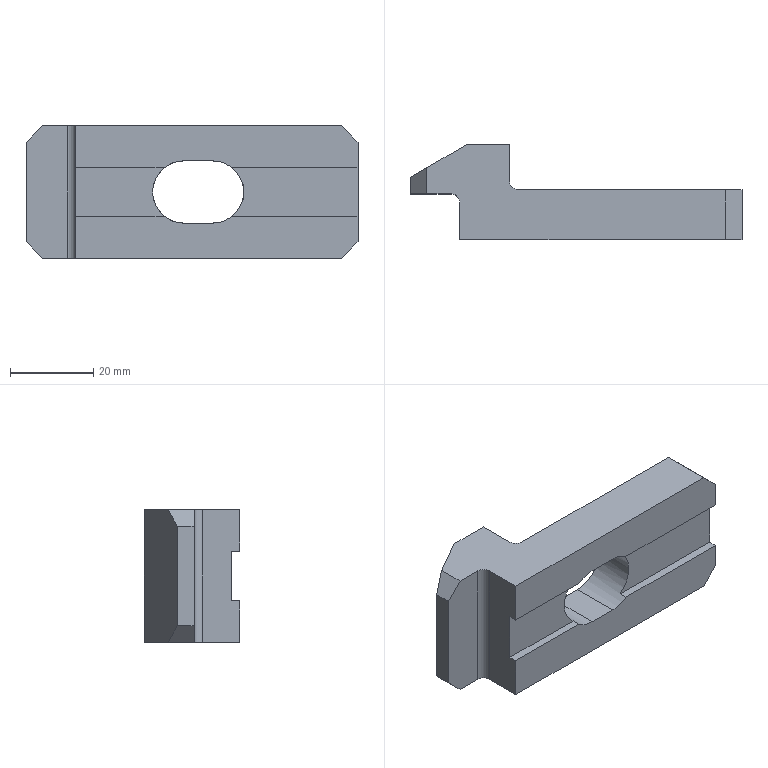Component | SolidWorks | JB_T8010.10-1999ElbowClampPlateTypeA12-1 | 1 solid | 28 faces | box 80 x 23 x 32 mm | volume 28429 mm3 | plane 24 | cylinder 4 | commonest cylinder face diameters 15 x2 4 x2 | material Nickel
STEP:
#1=COLOUR_RGB('',0.7922,0.8196,0.9333);
#2=FILL_AREA_STYLE_COLOUR('',#1);
#3=FILL_AREA_STYLE('',(#2));
#4=SURFACE_STYLE_FILL_AREA(#3);
#5=SURFACE_SIDE_STYLE('',(#4));
#6=SURFACE_STYLE_USAGE(.BOTH.,#5);
#7=PRESENTATION_STYLE_ASSIGNMENT((#6));
#8=CARTESIAN_POINT('',(2.48,8.528,-0.2362));
#9=VERTEX_POINT('',#8);
#10=CARTESIAN_POINT('',(3.327,8.528,-0.2362));
#11=VERTEX_POINT('',#10);
#12=CARTESIAN_POINT('',(2.008,8.528,-0.2362));
#13=DIRECTION('',(1.,0.,0.));
#14=VECTOR('',#13,39.37);
#15=LINE('',#12,#14);
#16=EDGE_CURVE('',#9,#11,#15,.T.);
#17=ORIENTED_EDGE('',*,*,#16,.F.);
#18=CARTESIAN_POINT('',(2.48,8.528,-0.6299));
#19=VERTEX_POINT('',#18);
#20=CARTESIAN_POINT('',(2.48,8.528,0.6299));
#21=DIRECTION('',(-0.,0.,-1.));
#22=VECTOR('',#21,39.37);
#23=LINE('',#20,#22);
#24=EDGE_CURVE('',#9,#19,#23,.T.);
#25=ORIENTED_EDGE('',*,*,#24,.T.);
#26=CARTESIAN_POINT('',(5.,8.528,-0.6299));
#27=VERTEX_POINT('',#26);
#28=CARTESIAN_POINT('',(2.48,8.528,-0.6299));
#29=DIRECTION('',(1.,0.,0.));
#30=VECTOR('',#29,39.37);
#31=LINE('',#28,#30);
#32=EDGE_CURVE('',#19,#27,#31,.T.);
#33=ORIENTED_EDGE('',*,*,#32,.T.);
#34=CARTESIAN_POINT('',(5.157,8.528,-0.4724));
#35=VERTEX_POINT('',#34);
#36=CARTESIAN_POINT('',(3.819,8.528,-1.811));
#37=DIRECTION('',(0.7071,0.,0.7071));
#38=VECTOR('',#37,39.37);
#39=LINE('',#36,#38);
#40=EDGE_CURVE('',#27,#35,#39,.T.);
#41=ORIENTED_EDGE('',*,*,#40,.T.);
#42=CARTESIAN_POINT('',(5.157,8.528,-0.2362));
#43=VERTEX_POINT('',#42);
#44=CARTESIAN_POINT('',(5.157,8.528,-0.6299));
#45=DIRECTION('',(0.,0.,1.));
#46=VECTOR('',#45,39.37);
#47=LINE('',#44,#46);
#48=EDGE_CURVE('',#35,#43,#47,.T.);
#49=ORIENTED_EDGE('',*,*,#48,.T.);
#50=CARTESIAN_POINT('',(3.957,8.528,-0.2362));
#51=VERTEX_POINT('',#50);
#52=CARTESIAN_POINT('',(2.008,8.528,-0.2362));
#53=DIRECTION('',(1.,0.,0.));
#54=VECTOR('',#53,39.37);
#55=LINE('',#52,#54);
#56=EDGE_CURVE('',#51,#43,#55,.T.);
#57=ORIENTED_EDGE('',*,*,#56,.F.);
#58=CARTESIAN_POINT('',(3.78,8.528,-0.2953));
#59=VERTEX_POINT('',#58);
#60=CARTESIAN_POINT('',(3.78,8.528,0.));
#61=DIRECTION('',(0.,-1.,0.));
#62=DIRECTION('',(0.,0.,-1.));
#63=AXIS2_PLACEMENT_3D('',#60,#61,#62);
#64=CIRCLE('',#63,0.2953);
#65=EDGE_CURVE('',#59,#51,#64,.T.);
#66=ORIENTED_EDGE('',*,*,#65,.F.);
#67=CARTESIAN_POINT('',(3.504,8.528,-0.2953));
#68=VERTEX_POINT('',#67);
#69=CARTESIAN_POINT('',(3.504,8.528,-0.2953));
#70=DIRECTION('',(1.,0.,0.));
#71=VECTOR('',#70,39.37);
#72=LINE('',#69,#71);
#73=EDGE_CURVE('',#68,#59,#72,.T.);
#74=ORIENTED_EDGE('',*,*,#73,.F.);
#75=CARTESIAN_POINT('',(3.504,8.528,0.));
#76=DIRECTION('',(0.,-1.,0.));
#77=DIRECTION('',(0.,0.,-1.));
#78=AXIS2_PLACEMENT_3D('',#75,#76,#77);
#79=CIRCLE('',#78,0.2953);
#80=EDGE_CURVE('',#11,#68,#79,.T.);
#81=ORIENTED_EDGE('',*,*,#80,.F.);
#82=EDGE_LOOP('',(#17,#25,#33,#41,#49,#57,#66,#74,#81));
#83=FACE_OUTER_BOUND('',#82,.T.);
#84=CARTESIAN_POINT('',(2.008,8.528,0.));
#85=DIRECTION('',(0.,-1.,0.));
#86=DIRECTION('',(0.,0.,-1.));
#87=AXIS2_PLACEMENT_3D('',#84,#85,#86);
#88=PLANE('',#87);
#89=ADVANCED_FACE('',(#83),#88,.T.);
#90=CARTESIAN_POINT('',(5.,9.,-0.6299));
#91=VERTEX_POINT('',#90);
#92=CARTESIAN_POINT('',(3.031,9.,-0.6299));
#93=VERTEX_POINT('',#92);
#94=CARTESIAN_POINT('',(5.157,9.,-0.6299));
#95=DIRECTION('',(-1.,0.,0.));
#96=VECTOR('',#95,39.37);
#97=LINE('',#94,#96);
#98=EDGE_CURVE('',#91,#93,#97,.T.);
#99=ORIENTED_EDGE('',*,*,#98,.F.);
#100=CARTESIAN_POINT('',(5.,8.803,-0.6299));
#101=DIRECTION('',(0.,-1.,0.));
#102=VECTOR('',#101,39.37);
#103=LINE('',#100,#102);
#104=EDGE_CURVE('',#91,#27,#103,.T.);
#105=ORIENTED_EDGE('',*,*,#104,.T.);
#106=ORIENTED_EDGE('',*,*,#32,.F.);
#107=CARTESIAN_POINT('',(2.48,8.882,-0.6299));
#108=VERTEX_POINT('',#107);
#109=CARTESIAN_POINT('',(2.48,8.961,-0.6299));
#110=DIRECTION('',(0.,-1.,0.));
#111=VECTOR('',#110,39.37);
#112=LINE('',#109,#111);
#113=EDGE_CURVE('',#108,#19,#112,.T.);
#114=ORIENTED_EDGE('',*,*,#113,.F.);
#115=CARTESIAN_POINT('',(2.402,8.961,-0.6299));
#116=VERTEX_POINT('',#115);
#117=CARTESIAN_POINT('',(2.402,8.882,-0.6299));
#118=DIRECTION('',(0.,0.,1.));
#119=DIRECTION('',(1.,0.,0.));
#120=AXIS2_PLACEMENT_3D('',#117,#118,#119);
#121=CIRCLE('',#120,0.07874);
#122=EDGE_CURVE('',#108,#116,#121,.T.);
#123=ORIENTED_EDGE('',*,*,#122,.T.);
#124=CARTESIAN_POINT('',(2.165,8.961,-0.6299));
#125=VERTEX_POINT('',#124);
#126=CARTESIAN_POINT('',(2.008,8.961,-0.6299));
#127=DIRECTION('',(1.,0.,0.));
#128=VECTOR('',#127,39.37);
#129=LINE('',#126,#128);
#130=EDGE_CURVE('',#125,#116,#129,.T.);
#131=ORIENTED_EDGE('',*,*,#130,.F.);
#132=CARTESIAN_POINT('',(2.165,9.209,-0.6299));
#133=VERTEX_POINT('',#132);
#134=CARTESIAN_POINT('',(2.165,8.803,-0.6299));
#135=DIRECTION('',(0.,1.,0.));
#136=VECTOR('',#135,39.37);
#137=LINE('',#134,#136);
#138=EDGE_CURVE('',#125,#133,#137,.T.);
#139=ORIENTED_EDGE('',*,*,#138,.T.);
#140=CARTESIAN_POINT('',(2.553,9.433,-0.6299));
#141=VERTEX_POINT('',#140);
#142=CARTESIAN_POINT('',(1.871,9.04,-0.6299));
#143=DIRECTION('',(0.866,0.5,0.));
#144=VECTOR('',#143,39.37);
#145=LINE('',#142,#144);
#146=EDGE_CURVE('',#133,#141,#145,.T.);
#147=ORIENTED_EDGE('',*,*,#146,.T.);
#148=CARTESIAN_POINT('',(2.953,9.433,-0.6299));
#149=VERTEX_POINT('',#148);
#150=CARTESIAN_POINT('',(2.953,9.433,-0.6299));
#151=DIRECTION('',(-1.,0.,0.));
#152=VECTOR('',#151,39.37);
#153=LINE('',#150,#152);
#154=EDGE_CURVE('',#149,#141,#153,.T.);
#155=ORIENTED_EDGE('',*,*,#154,.F.);
#156=CARTESIAN_POINT('',(2.953,9.079,-0.6299));
#157=VERTEX_POINT('',#156);
#158=CARTESIAN_POINT('',(2.953,9.433,-0.6299));
#159=DIRECTION('',(0.,-1.,0.));
#160=VECTOR('',#159,39.37);
#161=LINE('',#158,#160);
#162=EDGE_CURVE('',#149,#157,#161,.T.);
#163=ORIENTED_EDGE('',*,*,#162,.T.);
#164=CARTESIAN_POINT('',(3.031,9.079,-0.6299));
#165=DIRECTION('',(0.,0.,1.));
#166=DIRECTION('',(1.,0.,0.));
#167=AXIS2_PLACEMENT_3D('',#164,#165,#166);
#168=CIRCLE('',#167,0.07874);
#169=EDGE_CURVE('',#157,#93,#168,.T.);
#170=ORIENTED_EDGE('',*,*,#169,.T.);
#171=EDGE_LOOP('',(#99,#105,#106,#114,#123,#131,#139,#147,#155,#163,#170));
#172=FACE_OUTER_BOUND('',#171,.T.);
#173=CARTESIAN_POINT('',(2.008,8.803,-0.6299));
#174=DIRECTION('',(0.,0.,1.));
#175=DIRECTION('',(1.,0.,0.));
#176=AXIS2_PLACEMENT_3D('',#173,#174,#175);
#177=PLANE('',#176);
#178=ADVANCED_FACE('',(#172),#177,.F.);
#179=CARTESIAN_POINT('',(2.553,9.433,0.6299));
#180=VERTEX_POINT('',#179);
#181=CARTESIAN_POINT('',(2.165,9.209,0.6299));
#182=VERTEX_POINT('',#181);
#183=CARTESIAN_POINT('',(1.871,9.04,0.6299));
#184=DIRECTION('',(-0.866,-0.5,0.));
#185=VECTOR('',#184,39.37);
#186=LINE('',#183,#185);
#187=EDGE_CURVE('',#180,#182,#186,.T.);
#188=ORIENTED_EDGE('',*,*,#187,.T.);
#189=CARTESIAN_POINT('',(2.165,8.961,0.6299));
#190=VERTEX_POINT('',#189);
#191=CARTESIAN_POINT('',(2.165,8.803,0.6299));
#192=DIRECTION('',(0.,-1.,0.));
#193=VECTOR('',#192,39.37);
#194=LINE('',#191,#193);
#195=EDGE_CURVE('',#182,#190,#194,.T.);
#196=ORIENTED_EDGE('',*,*,#195,.T.);
#197=CARTESIAN_POINT('',(2.402,8.961,0.6299));
#198=VERTEX_POINT('',#197);
#199=CARTESIAN_POINT('',(2.48,8.961,0.6299));
#200=DIRECTION('',(-1.,0.,0.));
#201=VECTOR('',#200,39.37);
#202=LINE('',#199,#201);
#203=EDGE_CURVE('',#198,#190,#202,.T.);
#204=ORIENTED_EDGE('',*,*,#203,.F.);
#205=CARTESIAN_POINT('',(2.48,8.882,0.6299));
#206=VERTEX_POINT('',#205);
#207=CARTESIAN_POINT('',(2.402,8.882,0.6299));
#208=DIRECTION('',(0.,0.,-1.));
#209=DIRECTION('',(-1.,0.,0.));
#210=AXIS2_PLACEMENT_3D('',#207,#208,#209);
#211=CIRCLE('',#210,0.07874);
#212=EDGE_CURVE('',#198,#206,#211,.T.);
#213=ORIENTED_EDGE('',*,*,#212,.T.);
#214=CARTESIAN_POINT('',(2.48,8.528,0.6299));
#215=VERTEX_POINT('',#214);
#216=CARTESIAN_POINT('',(2.48,8.961,0.6299));
#217=DIRECTION('',(0.,-1.,0.));
#218=VECTOR('',#217,39.37);
#219=LINE('',#216,#218);
#220=EDGE_CURVE('',#206,#215,#219,.T.);
#221=ORIENTED_EDGE('',*,*,#220,.T.);
#222=CARTESIAN_POINT('',(5.,8.528,0.6299));
#223=VERTEX_POINT('',#222);
#224=CARTESIAN_POINT('',(5.157,8.528,0.6299));
#225=DIRECTION('',(-1.,0.,0.));
#226=VECTOR('',#225,39.37);
#227=LINE('',#224,#226);
#228=EDGE_CURVE('',#223,#215,#227,.T.);
#229=ORIENTED_EDGE('',*,*,#228,.F.);
#230=CARTESIAN_POINT('',(5.,9.,0.6299));
#231=VERTEX_POINT('',#230);
#232=CARTESIAN_POINT('',(5.,8.803,0.6299));
#233=DIRECTION('',(0.,1.,0.));
#234=VECTOR('',#233,39.37);
#235=LINE('',#232,#234);
#236=EDGE_CURVE('',#223,#231,#235,.T.);
#237=ORIENTED_EDGE('',*,*,#236,.T.);
#238=CARTESIAN_POINT('',(3.031,9.,0.6299));
#239=VERTEX_POINT('',#238);
#240=CARTESIAN_POINT('',(5.157,9.,0.6299));
#241=DIRECTION('',(1.,0.,0.));
#242=VECTOR('',#241,39.37);
#243=LINE('',#240,#242);
#244=EDGE_CURVE('',#239,#231,#243,.T.);
#245=ORIENTED_EDGE('',*,*,#244,.F.);
#246=CARTESIAN_POINT('',(2.953,9.079,0.6299));
#247=VERTEX_POINT('',#246);
#248=CARTESIAN_POINT('',(3.031,9.079,0.6299));
#249=DIRECTION('',(0.,0.,-1.));
#250=DIRECTION('',(-1.,0.,0.));
#251=AXIS2_PLACEMENT_3D('',#248,#249,#250);
#252=CIRCLE('',#251,0.07874);
#253=EDGE_CURVE('',#239,#247,#252,.T.);
#254=ORIENTED_EDGE('',*,*,#253,.T.);
#255=CARTESIAN_POINT('',(2.953,9.433,0.6299));
#256=VERTEX_POINT('',#255);
#257=CARTESIAN_POINT('',(2.953,9.433,0.6299));
#258=DIRECTION('',(0.,-1.,0.));
#259=VECTOR('',#258,39.37);
#260=LINE('',#257,#259);
#261=EDGE_CURVE('',#256,#247,#260,.T.);
#262=ORIENTED_EDGE('',*,*,#261,.F.);
#263=CARTESIAN_POINT('',(2.008,9.433,0.6299));
#264=DIRECTION('',(1.,0.,0.));
#265=VECTOR('',#264,39.37);
#266=LINE('',#263,#265);
#267=EDGE_CURVE('',#180,#256,#266,.T.);
#268=ORIENTED_EDGE('',*,*,#267,.F.);
#269=EDGE_LOOP('',(#188,#196,#204,#213,#221,#229,#237,#245,#254,#262,#268));
#270=FACE_OUTER_BOUND('',#269,.T.);
#271=CARTESIAN_POINT('',(2.008,8.803,0.6299));
#272=DIRECTION('',(0.,0.,-1.));
#273=DIRECTION('',(-1.,0.,0.));
#274=AXIS2_PLACEMENT_3D('',#271,#272,#273);
#275=PLANE('',#274);
#276=ADVANCED_FACE('',(#270),#275,.F.);
#277=CARTESIAN_POINT('',(5.157,8.607,-0.2362));
#278=VERTEX_POINT('',#277);
#279=CARTESIAN_POINT('',(5.157,8.607,0.2362));
#280=VERTEX_POINT('',#279);
#281=CARTESIAN_POINT('',(5.157,8.607,-0.6299));
#282=DIRECTION('',(0.,0.,1.));
#283=VECTOR('',#282,39.37);
#284=LINE('',#281,#283);
#285=EDGE_CURVE('',#278,#280,#284,.T.);
#286=ORIENTED_EDGE('',*,*,#285,.F.);
#287=CARTESIAN_POINT('',(5.157,8.803,-0.2362));
#288=DIRECTION('',(0.,-1.,0.));
#289=VECTOR('',#288,39.37);
#290=LINE('',#287,#289);
#291=EDGE_CURVE('',#278,#43,#290,.T.);
#292=ORIENTED_EDGE('',*,*,#291,.T.);
#293=ORIENTED_EDGE('',*,*,#48,.F.);
#294=CARTESIAN_POINT('',(5.157,9.,-0.4724));
#295=VERTEX_POINT('',#294);
#296=CARTESIAN_POINT('',(5.157,8.803,-0.4724));
#297=DIRECTION('',(0.,1.,0.));
#298=VECTOR('',#297,39.37);
#299=LINE('',#296,#298);
#300=EDGE_CURVE('',#35,#295,#299,.T.);
#301=ORIENTED_EDGE('',*,*,#300,.T.);
#302=CARTESIAN_POINT('',(5.157,9.,0.4724));
#303=VERTEX_POINT('',#302);
#304=CARTESIAN_POINT('',(5.157,9.,-0.6299));
#305=DIRECTION('',(0.,0.,-1.));
#306=VECTOR('',#305,39.37);
#307=LINE('',#304,#306);
#308=EDGE_CURVE('',#303,#295,#307,.T.);
#309=ORIENTED_EDGE('',*,*,#308,.F.);
#310=CARTESIAN_POINT('',(5.157,8.528,0.4724));
#311=VERTEX_POINT('',#310);
#312=CARTESIAN_POINT('',(5.157,8.803,0.4724));
#313=DIRECTION('',(0.,-1.,0.));
#314=VECTOR('',#313,39.37);
#315=LINE('',#312,#314);
#316=EDGE_CURVE('',#303,#311,#315,.T.);
#317=ORIENTED_EDGE('',*,*,#316,.T.);
#318=CARTESIAN_POINT('',(5.157,8.528,0.2362));
#319=VERTEX_POINT('',#318);
#320=CARTESIAN_POINT('',(5.157,8.528,-0.6299));
#321=DIRECTION('',(0.,0.,1.));
#322=VECTOR('',#321,39.37);
#323=LINE('',#320,#322);
#324=EDGE_CURVE('',#319,#311,#323,.T.);
#325=ORIENTED_EDGE('',*,*,#324,.F.);
#326=CARTESIAN_POINT('',(5.157,8.803,0.2362));
#327=DIRECTION('',(0.,1.,0.));
#328=VECTOR('',#327,39.37);
#329=LINE('',#326,#328);
#330=EDGE_CURVE('',#319,#280,#329,.T.);
#331=ORIENTED_EDGE('',*,*,#330,.T.);
#332=EDGE_LOOP('',(#286,#292,#293,#301,#309,#317,#325,#331));
#333=FACE_OUTER_BOUND('',#332,.T.);
#334=CARTESIAN_POINT('',(5.157,8.803,-0.6299));
#335=DIRECTION('',(-1.,0.,0.));
#336=DIRECTION('',(0.,0.,1.));
#337=AXIS2_PLACEMENT_3D('',#334,#335,#336);
#338=PLANE('',#337);
#339=ADVANCED_FACE('',(#333),#338,.F.);
#340=CARTESIAN_POINT('',(3.327,8.607,-0.2362));
#341=VERTEX_POINT('',#340);
#342=CARTESIAN_POINT('',(3.327,8.803,-0.2362));
#343=DIRECTION('',(0.,1.,0.));
#344=VECTOR('',#343,39.37);
#345=LINE('',#342,#344);
#346=EDGE_CURVE('',#11,#341,#345,.T.);
#347=ORIENTED_EDGE('',*,*,#346,.F.);
#348=ORIENTED_EDGE('',*,*,#80,.T.);
#349=CARTESIAN_POINT('',(3.504,9.,-0.2953));
#350=VERTEX_POINT('',#349);
#351=CARTESIAN_POINT('',(3.504,8.803,-0.2953));
#352=DIRECTION('',(0.,-1.,0.));
#353=VECTOR('',#352,39.37);
#354=LINE('',#351,#353);
#355=EDGE_CURVE('',#350,#68,#354,.T.);
#356=ORIENTED_EDGE('',*,*,#355,.F.);
#357=CARTESIAN_POINT('',(3.504,9.,0.2953));
#358=VERTEX_POINT('',#357);
#359=CARTESIAN_POINT('',(3.504,9.,0.));
#360=DIRECTION('',(0.,1.,0.));
#361=DIRECTION('',(0.,0.,-1.));
#362=AXIS2_PLACEMENT_3D('',#359,#360,#361);
#363=CIRCLE('',#362,0.2953);
#364=EDGE_CURVE('',#350,#358,#363,.T.);
#365=ORIENTED_EDGE('',*,*,#364,.T.);
#366=CARTESIAN_POINT('',(3.504,8.528,0.2953));
#367=VERTEX_POINT('',#366);
#368=CARTESIAN_POINT('',(3.504,8.803,0.2953));
#369=DIRECTION('',(0.,-1.,0.));
#370=VECTOR('',#369,39.37);
#371=LINE('',#368,#370);
#372=EDGE_CURVE('',#358,#367,#371,.T.);
#373=ORIENTED_EDGE('',*,*,#372,.T.);
#374=CARTESIAN_POINT('',(3.327,8.528,0.2362));
#375=VERTEX_POINT('',#374);
#376=CARTESIAN_POINT('',(3.504,8.528,0.));
#377=DIRECTION('',(0.,-1.,0.));
#378=DIRECTION('',(0.,0.,-1.));
#379=AXIS2_PLACEMENT_3D('',#376,#377,#378);
#380=CIRCLE('',#379,0.2953);
#381=EDGE_CURVE('',#367,#375,#380,.T.);
#382=ORIENTED_EDGE('',*,*,#381,.T.);
#383=CARTESIAN_POINT('',(3.327,8.607,0.2362));
#384=VERTEX_POINT('',#383);
#385=CARTESIAN_POINT('',(3.327,8.803,0.2362));
#386=DIRECTION('',(0.,-1.,0.));
#387=VECTOR('',#386,39.37);
#388=LINE('',#385,#387);
#389=EDGE_CURVE('',#384,#375,#388,.T.);
#390=ORIENTED_EDGE('',*,*,#389,.F.);
#391=CARTESIAN_POINT('',(3.504,8.607,0.));
#392=DIRECTION('',(0.,-1.,0.));
#393=DIRECTION('',(0.,0.,-1.));
#394=AXIS2_PLACEMENT_3D('',#391,#392,#393);
#395=CIRCLE('',#394,0.2953);
#396=EDGE_CURVE('',#384,#341,#395,.T.);
#397=ORIENTED_EDGE('',*,*,#396,.T.);
#398=EDGE_LOOP('',(#347,#348,#356,#365,#373,#382,#390,#397));
#399=FACE_OUTER_BOUND('',#398,.T.);
#400=CARTESIAN_POINT('',(3.504,8.803,0.));
#401=DIRECTION('',(0.,-1.,0.));
#402=DIRECTION('',(0.,0.,-1.));
#403=AXIS2_PLACEMENT_3D('',#400,#401,#402);
#404=CYLINDRICAL_SURFACE('',#403,0.2953);
#405=ADVANCED_FACE('',(#399),#404,.F.);
#406=CARTESIAN_POINT('',(3.78,9.,0.2953));
#407=VERTEX_POINT('',#406);
#408=CARTESIAN_POINT('',(3.78,8.528,0.2953));
#409=VERTEX_POINT('',#408);
#410=CARTESIAN_POINT('',(3.78,8.803,0.2953));
#411=DIRECTION('',(0.,-1.,0.));
#412=VECTOR('',#411,39.37);
#413=LINE('',#410,#412);
#414=EDGE_CURVE('',#407,#409,#413,.T.);
#415=ORIENTED_EDGE('',*,*,#414,.T.);
#416=CARTESIAN_POINT('',(3.504,8.528,0.2953));
#417=DIRECTION('',(-1.,0.,0.));
#418=VECTOR('',#417,39.37);
#419=LINE('',#416,#418);
#420=EDGE_CURVE('',#409,#367,#419,.T.);
#421=ORIENTED_EDGE('',*,*,#420,.T.);
#422=ORIENTED_EDGE('',*,*,#372,.F.);
#423=CARTESIAN_POINT('',(5.157,9.,0.2953));
#424=DIRECTION('',(1.,0.,0.));
#425=VECTOR('',#424,39.37);
#426=LINE('',#423,#425);
#427=EDGE_CURVE('',#358,#407,#426,.T.);
#428=ORIENTED_EDGE('',*,*,#427,.T.);
#429=EDGE_LOOP('',(#415,#421,#422,#428));
#430=FACE_OUTER_BOUND('',#429,.T.);
#431=CARTESIAN_POINT('',(3.504,8.803,0.2953));
#432=DIRECTION('',(0.,0.,-1.));
#433=DIRECTION('',(-1.,0.,0.));
#434=AXIS2_PLACEMENT_3D('',#431,#432,#433);
#435=PLANE('',#434);
#436=ADVANCED_FACE('',(#430),#435,.T.);
#437=CARTESIAN_POINT('',(3.957,8.607,-0.2362));
#438=VERTEX_POINT('',#437);
#439=CARTESIAN_POINT('',(3.957,8.803,-0.2362));
#440=DIRECTION('',(0.,-1.,0.));
#441=VECTOR('',#440,39.37);
#442=LINE('',#439,#441);
#443=EDGE_CURVE('',#438,#51,#442,.T.);
#444=ORIENTED_EDGE('',*,*,#443,.F.);
#445=CARTESIAN_POINT('',(3.957,8.607,0.2362));
#446=VERTEX_POINT('',#445);
#447=CARTESIAN_POINT('',(3.78,8.607,0.));
#448=DIRECTION('',(0.,-1.,0.));
#449=DIRECTION('',(0.,0.,-1.));
#450=AXIS2_PLACEMENT_3D('',#447,#448,#449);
#451=CIRCLE('',#450,0.2953);
#452=EDGE_CURVE('',#438,#446,#451,.T.);
#453=ORIENTED_EDGE('',*,*,#452,.T.);
#454=CARTESIAN_POINT('',(3.957,8.528,0.2362));
#455=VERTEX_POINT('',#454);
#456=CARTESIAN_POINT('',(3.957,8.803,0.2362));
#457=DIRECTION('',(0.,1.,0.));
#458=VECTOR('',#457,39.37);
#459=LINE('',#456,#458);
#460=EDGE_CURVE('',#455,#446,#459,.T.);
#461=ORIENTED_EDGE('',*,*,#460,.F.);
#462=CARTESIAN_POINT('',(3.78,8.528,0.));
#463=DIRECTION('',(0.,-1.,0.));
#464=DIRECTION('',(0.,0.,-1.));
#465=AXIS2_PLACEMENT_3D('',#462,#463,#464);
#466=CIRCLE('',#465,0.2953);
#467=EDGE_CURVE('',#455,#409,#466,.T.);
#468=ORIENTED_EDGE('',*,*,#467,.T.);
#469=ORIENTED_EDGE('',*,*,#414,.F.);
#470=CARTESIAN_POINT('',(3.78,9.,-0.2953));
#471=VERTEX_POINT('',#470);
#472=CARTESIAN_POINT('',(3.78,9.,0.));
#473=DIRECTION('',(0.,1.,0.));
#474=DIRECTION('',(0.,0.,-1.));
#475=AXIS2_PLACEMENT_3D('',#472,#473,#474);
#476=CIRCLE('',#475,0.2953);
#477=EDGE_CURVE('',#407,#471,#476,.T.);
#478=ORIENTED_EDGE('',*,*,#477,.T.);
#479=CARTESIAN_POINT('',(3.78,8.803,-0.2953));
#480=DIRECTION('',(0.,-1.,0.));
#481=VECTOR('',#480,39.37);
#482=LINE('',#479,#481);
#483=EDGE_CURVE('',#471,#59,#482,.T.);
#484=ORIENTED_EDGE('',*,*,#483,.T.);
#485=ORIENTED_EDGE('',*,*,#65,.T.);
#486=EDGE_LOOP('',(#444,#453,#461,#468,#469,#478,#484,#485));
#487=FACE_OUTER_BOUND('',#486,.T.);
#488=CARTESIAN_POINT('',(3.78,8.803,0.));
#489=DIRECTION('',(0.,-1.,0.));
#490=DIRECTION('',(0.,0.,-1.));
#491=AXIS2_PLACEMENT_3D('',#488,#489,#490);
#492=CYLINDRICAL_SURFACE('',#491,0.2953);
#493=ADVANCED_FACE('',(#487),#492,.F.);
#494=ORIENTED_EDGE('',*,*,#355,.T.);
#495=ORIENTED_EDGE('',*,*,#73,.T.);
#496=ORIENTED_EDGE('',*,*,#483,.F.);
#497=CARTESIAN_POINT('',(5.157,9.,-0.2953));
#498=DIRECTION('',(-1.,0.,0.));
#499=VECTOR('',#498,39.37);
#500=LINE('',#497,#499);
#501=EDGE_CURVE('',#471,#350,#500,.T.);
#502=ORIENTED_EDGE('',*,*,#501,.T.);
#503=EDGE_LOOP('',(#494,#495,#496,#502));
#504=FACE_OUTER_BOUND('',#503,.T.);
#505=CARTESIAN_POINT('',(3.504,8.803,-0.2953));
#506=DIRECTION('',(0.,0.,1.));
#507=DIRECTION('',(1.,0.,0.));
#508=AXIS2_PLACEMENT_3D('',#505,#506,#507);
#509=PLANE('',#508);
#510=ADVANCED_FACE('',(#504),#509,.T.);
#511=ORIENTED_EDGE('',*,*,#24,.F.);
#512=CARTESIAN_POINT('',(2.48,8.607,-0.2362));
#513=VERTEX_POINT('',#512);
#514=CARTESIAN_POINT('',(2.48,8.961,-0.2362));
#515=DIRECTION('',(0.,1.,0.));
#516=VECTOR('',#515,39.37);
#517=LINE('',#514,#516);
#518=EDGE_CURVE('',#9,#513,#517,.T.);
#519=ORIENTED_EDGE('',*,*,#518,.T.);
#520=CARTESIAN_POINT('',(2.48,8.607,0.2362));
#521=VERTEX_POINT('',#520);
#522=CARTESIAN_POINT('',(2.48,8.607,-0.6299));
#523=DIRECTION('',(-0.,0.,-1.));
#524=VECTOR('',#523,39.37);
#525=LINE('',#522,#524);
#526=EDGE_CURVE('',#521,#513,#525,.T.);
#527=ORIENTED_EDGE('',*,*,#526,.F.);
#528=CARTESIAN_POINT('',(2.48,8.528,0.2362));
#529=VERTEX_POINT('',#528);
#530=CARTESIAN_POINT('',(2.48,8.961,0.2362));
#531=DIRECTION('',(0.,-1.,0.));
#532=VECTOR('',#531,39.37);
#533=LINE('',#530,#532);
#534=EDGE_CURVE('',#521,#529,#533,.T.);
#535=ORIENTED_EDGE('',*,*,#534,.T.);
#536=CARTESIAN_POINT('',(2.48,8.528,0.6299));
#537=DIRECTION('',(-0.,0.,-1.));
#538=VECTOR('',#537,39.37);
#539=LINE('',#536,#538);
#540=EDGE_CURVE('',#215,#529,#539,.T.);
#541=ORIENTED_EDGE('',*,*,#540,.F.);
#542=ORIENTED_EDGE('',*,*,#220,.F.);
#543=CARTESIAN_POINT('',(2.48,8.882,-0.6299));
#544=DIRECTION('',(-0.,0.,-1.));
#545=VECTOR('',#544,39.37);
#546=LINE('',#543,#545);
#547=EDGE_CURVE('',#206,#108,#546,.T.);
#548=ORIENTED_EDGE('',*,*,#547,.T.);
#549=ORIENTED_EDGE('',*,*,#113,.T.);
#550=EDGE_LOOP('',(#511,#519,#527,#535,#541,#542,#548,#549));
#551=FACE_OUTER_BOUND('',#550,.T.);
#552=CARTESIAN_POINT('',(2.48,8.961,-0.6299));
#553=DIRECTION('',(1.,0.,-0.));
#554=DIRECTION('',(-0.,0.,-1.));
#555=AXIS2_PLACEMENT_3D('',#552,#553,#554);
#556=PLANE('',#555);
#557=ADVANCED_FACE('',(#551),#556,.F.);
#558=CARTESIAN_POINT('',(2.008,8.961,0.4724));
#559=VERTEX_POINT('',#558);
#560=CARTESIAN_POINT('',(2.008,8.961,-0.4724));
#561=VERTEX_POINT('',#560);
#562=CARTESIAN_POINT('',(2.008,8.961,0.6299));
#563=DIRECTION('',(0.,0.,-1.));
#564=VECTOR('',#563,39.37);
#565=LINE('',#562,#564);
#566=EDGE_CURVE('',#559,#561,#565,.T.);
#567=ORIENTED_EDGE('',*,*,#566,.F.);
#568=CARTESIAN_POINT('',(2.008,9.118,0.4724));
#569=VERTEX_POINT('',#568);
#570=CARTESIAN_POINT('',(2.008,8.803,0.4724));
#571=DIRECTION('',(0.,1.,0.));
#572=VECTOR('',#571,39.37);
#573=LINE('',#570,#572);
#574=EDGE_CURVE('',#559,#569,#573,.T.);
#575=ORIENTED_EDGE('',*,*,#574,.T.);
#576=CARTESIAN_POINT('',(2.008,9.118,-0.4724));
#577=VERTEX_POINT('',#576);
#578=CARTESIAN_POINT('',(2.008,9.118,-0.6299));
#579=DIRECTION('',(0.,0.,1.));
#580=VECTOR('',#579,39.37);
#581=LINE('',#578,#580);
#582=EDGE_CURVE('',#577,#569,#581,.T.);
#583=ORIENTED_EDGE('',*,*,#582,.F.);
#584=CARTESIAN_POINT('',(2.008,8.803,-0.4724));
#585=DIRECTION('',(0.,-1.,0.));
#586=VECTOR('',#585,39.37);
#587=LINE('',#584,#586);
#588=EDGE_CURVE('',#577,#561,#587,.T.);
#589=ORIENTED_EDGE('',*,*,#588,.T.);
#590=EDGE_LOOP('',(#567,#575,#583,#589));
#591=FACE_OUTER_BOUND('',#590,.T.);
#592=CARTESIAN_POINT('',(2.008,8.803,0.6299));
#593=DIRECTION('',(1.,0.,0.));
#594=DIRECTION('',(0.,0.,-1.));
#595=AXIS2_PLACEMENT_3D('',#592,#593,#594);
#596=PLANE('',#595);
#597=ADVANCED_FACE('',(#591),#596,.F.);
#598=ORIENTED_EDGE('',*,*,#364,.F.);
#599=ORIENTED_EDGE('',*,*,#501,.F.);
#600=ORIENTED_EDGE('',*,*,#477,.F.);
#601=ORIENTED_EDGE('',*,*,#427,.F.);
#602=EDGE_LOOP('',(#598,#599,#600,#601));
#603=FACE_BOUND('',#602,.T.);
#604=ORIENTED_EDGE('',*,*,#244,.T.);
#605=CARTESIAN_POINT('',(5.157,9.,0.4724));
#606=DIRECTION('',(0.7071,0.,-0.7071));
#607=VECTOR('',#606,39.37);
#608=LINE('',#605,#607);
#609=EDGE_CURVE('',#231,#303,#608,.T.);
#610=ORIENTED_EDGE('',*,*,#609,.T.);
#611=ORIENTED_EDGE('',*,*,#308,.T.);
#612=CARTESIAN_POINT('',(5.,9.,-0.6299));
#613=DIRECTION('',(-0.7071,0.,-0.7071));
#614=VECTOR('',#613,39.37);
#615=LINE('',#612,#614);
#616=EDGE_CURVE('',#295,#91,#615,.T.);
#617=ORIENTED_EDGE('',*,*,#616,.T.);
#618=ORIENTED_EDGE('',*,*,#98,.T.);
#619=CARTESIAN_POINT('',(3.031,9.,0.6299));
#620=DIRECTION('',(0.,0.,1.));
#621=VECTOR('',#620,39.37);
#622=LINE('',#619,#621);
#623=EDGE_CURVE('',#93,#239,#622,.T.);
#624=ORIENTED_EDGE('',*,*,#623,.T.);
#625=EDGE_LOOP('',(#604,#610,#611,#617,#618,#624));
#626=FACE_OUTER_BOUND('',#625,.T.);
#627=CARTESIAN_POINT('',(5.157,9.,-0.6299));
#628=DIRECTION('',(0.,-1.,0.));
#629=DIRECTION('',(0.,0.,-1.));
#630=AXIS2_PLACEMENT_3D('',#627,#628,#629);
#631=PLANE('',#630);
#632=ADVANCED_FACE('',(#603,#626),#631,.F.);
#633=ORIENTED_EDGE('',*,*,#261,.T.);
#634=CARTESIAN_POINT('',(2.953,9.079,-0.6299));
#635=DIRECTION('',(-0.,0.,-1.));
#636=VECTOR('',#635,39.37);
#637=LINE('',#634,#636);
#638=EDGE_CURVE('',#247,#157,#637,.T.);
#639=ORIENTED_EDGE('',*,*,#638,.T.);
#640=ORIENTED_EDGE('',*,*,#162,.F.);
#641=CARTESIAN_POINT('',(2.953,9.433,0.6299));
#642=DIRECTION('',(-0.,0.,-1.));
#643=VECTOR('',#642,39.37);
#644=LINE('',#641,#643);
#645=EDGE_CURVE('',#256,#149,#644,.T.);
#646=ORIENTED_EDGE('',*,*,#645,.F.);
#647=EDGE_LOOP('',(#633,#639,#640,#646));
#648=FACE_OUTER_BOUND('',#647,.T.);
#649=CARTESIAN_POINT('',(2.953,9.433,0.6299));
#650=DIRECTION('',(-1.,0.,0.));
#651=DIRECTION('',(0.,0.,1.));
#652=AXIS2_PLACEMENT_3D('',#649,#650,#651);
#653=PLANE('',#652);
#654=ADVANCED_FACE('',(#648),#653,.F.);
#655=CARTESIAN_POINT('',(2.553,9.433,-0.6299));
#656=DIRECTION('',(0.,0.,-1.));
#657=VECTOR('',#656,39.37);
#658=LINE('',#655,#657);
#659=EDGE_CURVE('',#180,#141,#658,.T.);
#660=ORIENTED_EDGE('',*,*,#659,.F.);
#661=ORIENTED_EDGE('',*,*,#267,.T.);
#662=ORIENTED_EDGE('',*,*,#645,.T.);
#663=ORIENTED_EDGE('',*,*,#154,.T.);
#664=EDGE_LOOP('',(#660,#661,#662,#663));
#665=FACE_OUTER_BOUND('',#664,.T.);
#666=CARTESIAN_POINT('',(2.008,9.433,-0.6299));
#667=DIRECTION('',(0.,1.,0.));
#668=DIRECTION('',(0.,0.,1.));
#669=AXIS2_PLACEMENT_3D('',#666,#667,#668);
#670=PLANE('',#669);
#671=ADVANCED_FACE('',(#665),#670,.T.);
#672=ORIENTED_EDGE('',*,*,#203,.T.);
#673=CARTESIAN_POINT('',(2.087,8.961,0.5512));
#674=DIRECTION('',(-0.7071,0.,-0.7071));
#675=VECTOR('',#674,39.37);
#676=LINE('',#673,#675);
#677=EDGE_CURVE('',#190,#559,#676,.T.);
#678=ORIENTED_EDGE('',*,*,#677,.T.);
#679=ORIENTED_EDGE('',*,*,#566,.T.);
#680=CARTESIAN_POINT('',(1.457,8.961,0.07874));
#681=DIRECTION('',(0.7071,0.,-0.7071));
#682=VECTOR('',#681,39.37);
#683=LINE('',#680,#682);
#684=EDGE_CURVE('',#561,#125,#683,.T.);
#685=ORIENTED_EDGE('',*,*,#684,.T.);
#686=ORIENTED_EDGE('',*,*,#130,.T.);
#687=CARTESIAN_POINT('',(2.402,8.961,0.6299));
#688=DIRECTION('',(0.,0.,1.));
#689=VECTOR('',#688,39.37);
#690=LINE('',#687,#689);
#691=EDGE_CURVE('',#116,#198,#690,.T.);
#692=ORIENTED_EDGE('',*,*,#691,.T.);
#693=EDGE_LOOP('',(#672,#678,#679,#685,#686,#692));
#694=FACE_OUTER_BOUND('',#693,.T.);
#695=CARTESIAN_POINT('',(2.008,8.961,0.6299));
#696=DIRECTION('',(0.,-1.,0.));
#697=DIRECTION('',(0.,0.,-1.));
#698=AXIS2_PLACEMENT_3D('',#695,#696,#697);
#699=PLANE('',#698);
#700=ADVANCED_FACE('',(#694),#699,.T.);
#701=ORIENTED_EDGE('',*,*,#582,.T.);
#702=CARTESIAN_POINT('',(2.065,9.151,0.5295));
#703=DIRECTION('',(0.6547,0.378,0.6547));
#704=VECTOR('',#703,39.37);
#705=LINE('',#702,#704);
#706=EDGE_CURVE('',#569,#182,#705,.T.);
#707=ORIENTED_EDGE('',*,*,#706,.T.);
#708=ORIENTED_EDGE('',*,*,#187,.F.);
#709=ORIENTED_EDGE('',*,*,#659,.T.);
#710=ORIENTED_EDGE('',*,*,#146,.F.);
#711=CARTESIAN_POINT('',(1.93,9.073,-0.3945));
#712=DIRECTION('',(-0.6547,-0.378,0.6547));
#713=VECTOR('',#712,39.37);
#714=LINE('',#711,#713);
#715=EDGE_CURVE('',#133,#577,#714,.T.);
#716=ORIENTED_EDGE('',*,*,#715,.T.);
#717=EDGE_LOOP('',(#701,#707,#708,#709,#710,#716));
#718=FACE_OUTER_BOUND('',#717,.T.);
#719=CARTESIAN_POINT('',(2.008,9.118,-0.6299));
#720=DIRECTION('',(0.5,-0.866,0.));
#721=DIRECTION('',(0.866,0.5,0.));
#722=AXIS2_PLACEMENT_3D('',#719,#720,#721);
#723=PLANE('',#722);
#724=ADVANCED_FACE('',(#718),#723,.F.);
#725=CARTESIAN_POINT('',(2.008,8.528,0.2362));
#726=DIRECTION('',(-1.,0.,-0.));
#727=VECTOR('',#726,39.37);
#728=LINE('',#725,#727);
#729=EDGE_CURVE('',#319,#455,#728,.T.);
#730=ORIENTED_EDGE('',*,*,#729,.F.);
#731=ORIENTED_EDGE('',*,*,#324,.T.);
#732=CARTESIAN_POINT('',(3.819,8.528,1.811));
#733=DIRECTION('',(-0.7071,0.,0.7071));
#734=VECTOR('',#733,39.37);
#735=LINE('',#732,#734);
#736=EDGE_CURVE('',#311,#223,#735,.T.);
#737=ORIENTED_EDGE('',*,*,#736,.T.);
#738=ORIENTED_EDGE('',*,*,#228,.T.);
#739=ORIENTED_EDGE('',*,*,#540,.T.);
#740=CARTESIAN_POINT('',(2.008,8.528,0.2362));
#741=DIRECTION('',(-1.,0.,-0.));
#742=VECTOR('',#741,39.37);
#743=LINE('',#740,#742);
#744=EDGE_CURVE('',#375,#529,#743,.T.);
#745=ORIENTED_EDGE('',*,*,#744,.F.);
#746=ORIENTED_EDGE('',*,*,#381,.F.);
#747=ORIENTED_EDGE('',*,*,#420,.F.);
#748=ORIENTED_EDGE('',*,*,#467,.F.);
#749=EDGE_LOOP('',(#730,#731,#737,#738,#739,#745,#746,#747,#748));
#750=FACE_OUTER_BOUND('',#749,.T.);
#751=CARTESIAN_POINT('',(2.008,8.528,0.));
#752=DIRECTION('',(0.,-1.,0.));
#753=DIRECTION('',(0.,0.,-1.));
#754=AXIS2_PLACEMENT_3D('',#751,#752,#753);
#755=PLANE('',#754);
#756=ADVANCED_FACE('',(#750),#755,.T.);
#757=ORIENTED_EDGE('',*,*,#253,.F.);
#758=ORIENTED_EDGE('',*,*,#623,.F.);
#759=ORIENTED_EDGE('',*,*,#169,.F.);
#760=ORIENTED_EDGE('',*,*,#638,.F.);
#761=EDGE_LOOP('',(#757,#758,#759,#760));
#762=FACE_OUTER_BOUND('',#761,.T.);
#763=CARTESIAN_POINT('',(3.031,9.079,0.6299));
#764=DIRECTION('',(0.,0.,1.));
#765=DIRECTION('',(1.,0.,0.));
#766=AXIS2_PLACEMENT_3D('',#763,#764,#765);
#767=CYLINDRICAL_SURFACE('',#766,0.07874);
#768=ADVANCED_FACE('',(#762),#767,.F.);
#769=ORIENTED_EDGE('',*,*,#122,.F.);
#770=ORIENTED_EDGE('',*,*,#547,.F.);
#771=ORIENTED_EDGE('',*,*,#212,.F.);
#772=ORIENTED_EDGE('',*,*,#691,.F.);
#773=EDGE_LOOP('',(#769,#770,#771,#772));
#774=FACE_OUTER_BOUND('',#773,.T.);
#775=CARTESIAN_POINT('',(2.402,8.882,0.6299));
#776=DIRECTION('',(0.,0.,1.));
#777=DIRECTION('',(1.,0.,0.));
#778=AXIS2_PLACEMENT_3D('',#775,#776,#777);
#779=CYLINDRICAL_SURFACE('',#778,0.07874);
#780=ADVANCED_FACE('',(#774),#779,.F.);
#781=ORIENTED_EDGE('',*,*,#706,.F.);
#782=ORIENTED_EDGE('',*,*,#574,.F.);
#783=ORIENTED_EDGE('',*,*,#677,.F.);
#784=ORIENTED_EDGE('',*,*,#195,.F.);
#785=EDGE_LOOP('',(#781,#782,#783,#784));
#786=FACE_OUTER_BOUND('',#785,.T.);
#787=CARTESIAN_POINT('',(2.165,8.803,0.6299));
#788=DIRECTION('',(0.7071,0.,-0.7071));
#789=DIRECTION('',(-0.7071,0.,-0.7071));
#790=AXIS2_PLACEMENT_3D('',#787,#788,#789);
#791=PLANE('',#790);
#792=ADVANCED_FACE('',(#786),#791,.F.);
#793=ORIENTED_EDGE('',*,*,#609,.F.);
#794=ORIENTED_EDGE('',*,*,#236,.F.);
#795=ORIENTED_EDGE('',*,*,#736,.F.);
#796=ORIENTED_EDGE('',*,*,#316,.F.);
#797=EDGE_LOOP('',(#793,#794,#795,#796));
#798=FACE_OUTER_BOUND('',#797,.T.);
#799=CARTESIAN_POINT('',(5.157,8.803,0.4724));
#800=DIRECTION('',(-0.7071,0.,-0.7071));
#801=DIRECTION('',(-0.7071,0.,0.7071));
#802=AXIS2_PLACEMENT_3D('',#799,#800,#801);
#803=PLANE('',#802);
#804=ADVANCED_FACE('',(#798),#803,.F.);
#805=ORIENTED_EDGE('',*,*,#616,.F.);
#806=ORIENTED_EDGE('',*,*,#300,.F.);
#807=ORIENTED_EDGE('',*,*,#40,.F.);
#808=ORIENTED_EDGE('',*,*,#104,.F.);
#809=EDGE_LOOP('',(#805,#806,#807,#808));
#810=FACE_OUTER_BOUND('',#809,.T.);
#811=CARTESIAN_POINT('',(5.,8.803,-0.6299));
#812=DIRECTION('',(-0.7071,0.,0.7071));
#813=DIRECTION('',(0.7071,0.,0.7071));
#814=AXIS2_PLACEMENT_3D('',#811,#812,#813);
#815=PLANE('',#814);
#816=ADVANCED_FACE('',(#810),#815,.F.);
#817=ORIENTED_EDGE('',*,*,#715,.F.);
#818=ORIENTED_EDGE('',*,*,#138,.F.);
#819=ORIENTED_EDGE('',*,*,#684,.F.);
#820=ORIENTED_EDGE('',*,*,#588,.F.);
#821=EDGE_LOOP('',(#817,#818,#819,#820));
#822=FACE_OUTER_BOUND('',#821,.T.);
#823=CARTESIAN_POINT('',(2.008,8.803,-0.4724));
#824=DIRECTION('',(0.7071,0.,0.7071));
#825=DIRECTION('',(0.7071,0.,-0.7071));
#826=AXIS2_PLACEMENT_3D('',#823,#824,#825);
#827=PLANE('',#826);
#828=ADVANCED_FACE('',(#822),#827,.F.);
#829=ORIENTED_EDGE('',*,*,#346,.T.);
#830=CARTESIAN_POINT('',(-1.929,8.607,-0.2362));
#831=DIRECTION('',(1.,0.,0.));
#832=VECTOR('',#831,39.37);
#833=LINE('',#830,#832);
#834=EDGE_CURVE('',#513,#341,#833,.T.);
#835=ORIENTED_EDGE('',*,*,#834,.F.);
#836=ORIENTED_EDGE('',*,*,#518,.F.);
#837=ORIENTED_EDGE('',*,*,#16,.T.);
#838=EDGE_LOOP('',(#829,#835,#836,#837));
#839=FACE_OUTER_BOUND('',#838,.T.);
#840=CARTESIAN_POINT('',(-1.929,8.607,-0.2362));
#841=DIRECTION('',(0.,0.,-1.));
#842=DIRECTION('',(-1.,0.,-0.));
#843=AXIS2_PLACEMENT_3D('',#840,#841,#842);
#844=PLANE('',#843);
#845=ADVANCED_FACE('',(#839),#844,.F.);
#846=ORIENTED_EDGE('',*,*,#389,.T.);
#847=ORIENTED_EDGE('',*,*,#744,.T.);
#848=ORIENTED_EDGE('',*,*,#534,.F.);
#849=CARTESIAN_POINT('',(-1.929,8.607,0.2362));
#850=DIRECTION('',(-1.,0.,-0.));
#851=VECTOR('',#850,39.37);
#852=LINE('',#849,#851);
#853=EDGE_CURVE('',#384,#521,#852,.T.);
#854=ORIENTED_EDGE('',*,*,#853,.F.);
#855=EDGE_LOOP('',(#846,#847,#848,#854));
#856=FACE_OUTER_BOUND('',#855,.T.);
#857=CARTESIAN_POINT('',(-1.929,8.607,0.2362));
#858=DIRECTION('',(-0.,0.,1.));
#859=DIRECTION('',(1.,0.,0.));
#860=AXIS2_PLACEMENT_3D('',#857,#858,#859);
#861=PLANE('',#860);
#862=ADVANCED_FACE('',(#856),#861,.F.);
#863=ORIENTED_EDGE('',*,*,#853,.T.);
#864=ORIENTED_EDGE('',*,*,#526,.T.);
#865=ORIENTED_EDGE('',*,*,#834,.T.);
#866=ORIENTED_EDGE('',*,*,#396,.F.);
#867=EDGE_LOOP('',(#863,#864,#865,#866));
#868=FACE_OUTER_BOUND('',#867,.T.);
#869=CARTESIAN_POINT('',(2.008,8.607,0.));
#870=DIRECTION('',(0.,-1.,0.));
#871=DIRECTION('',(0.,0.,-1.));
#872=AXIS2_PLACEMENT_3D('',#869,#870,#871);
#873=PLANE('',#872);
#874=ADVANCED_FACE('',(#868),#873,.T.);
#875=ORIENTED_EDGE('',*,*,#285,.T.);
#876=CARTESIAN_POINT('',(-1.929,8.607,0.2362));
#877=DIRECTION('',(-1.,0.,-0.));
#878=VECTOR('',#877,39.37);
#879=LINE('',#876,#878);
#880=EDGE_CURVE('',#280,#446,#879,.T.);
#881=ORIENTED_EDGE('',*,*,#880,.T.);
#882=ORIENTED_EDGE('',*,*,#452,.F.);
#883=CARTESIAN_POINT('',(-1.929,8.607,-0.2362));
#884=DIRECTION('',(1.,0.,0.));
#885=VECTOR('',#884,39.37);
#886=LINE('',#883,#885);
#887=EDGE_CURVE('',#438,#278,#886,.T.);
#888=ORIENTED_EDGE('',*,*,#887,.T.);
#889=EDGE_LOOP('',(#875,#881,#882,#888));
#890=FACE_OUTER_BOUND('',#889,.T.);
#891=CARTESIAN_POINT('',(2.008,8.607,0.));
#892=DIRECTION('',(0.,-1.,0.));
#893=DIRECTION('',(0.,0.,-1.));
#894=AXIS2_PLACEMENT_3D('',#891,#892,#893);
#895=PLANE('',#894);
#896=ADVANCED_FACE('',(#890),#895,.T.);
#897=ORIENTED_EDGE('',*,*,#887,.F.);
#898=ORIENTED_EDGE('',*,*,#443,.T.);
#899=ORIENTED_EDGE('',*,*,#56,.T.);
#900=ORIENTED_EDGE('',*,*,#291,.F.);
#901=EDGE_LOOP('',(#897,#898,#899,#900));
#902=FACE_OUTER_BOUND('',#901,.T.);
#903=CARTESIAN_POINT('',(-1.929,8.607,-0.2362));
#904=DIRECTION('',(0.,0.,-1.));
#905=DIRECTION('',(-1.,0.,-0.));
#906=AXIS2_PLACEMENT_3D('',#903,#904,#905);
#907=PLANE('',#906);
#908=ADVANCED_FACE('',(#902),#907,.F.);
#909=ORIENTED_EDGE('',*,*,#729,.T.);
#910=ORIENTED_EDGE('',*,*,#460,.T.);
#911=ORIENTED_EDGE('',*,*,#880,.F.);
#912=ORIENTED_EDGE('',*,*,#330,.F.);
#913=EDGE_LOOP('',(#909,#910,#911,#912));
#914=FACE_OUTER_BOUND('',#913,.T.);
#915=CARTESIAN_POINT('',(-1.929,8.607,0.2362));
#916=DIRECTION('',(-0.,0.,1.));
#917=DIRECTION('',(1.,0.,0.));
#918=AXIS2_PLACEMENT_3D('',#915,#916,#917);
#919=PLANE('',#918);
#920=ADVANCED_FACE('',(#914),#919,.F.);
#921=CLOSED_SHELL('',(#89,#178,#276,#339,#405,#436,#493,#510,#557,#597,#632,#654,#671,#700,#724,#756,#768,#780,#792,#804,#816,#828,#845,#862,#874,#896,#908,#920));
#922=MANIFOLD_SOLID_BREP('',#921);
#923=STYLED_ITEM('',(#7),#922);
#924=PRESENTATION_LAYER_ASSIGNMENT('','',(#923));
#925=CARTESIAN_POINT('',(0.,0.,0.));
#926=DIRECTION('',(0.,0.,1.));
#927=DIRECTION('',(1.,0.,0.));
#928=AXIS2_PLACEMENT_3D('',#925,#926,#927);
#929=(LENGTH_UNIT()NAMED_UNIT(*)SI_UNIT($,.METRE.));
#930=LENGTH_MEASURE_WITH_UNIT(LENGTH_MEASURE(0.0254),#929);
#931=DIMENSIONAL_EXPONENTS(1.,0.,0.,0.,0.,0.,0.);
#932=(CONVERSION_BASED_UNIT('',#930)LENGTH_UNIT()NAMED_UNIT(#931));
#933=UNCERTAINTY_MEASURE_WITH_UNIT(LENGTH_MEASURE(0.00001),#932,'','');
#934=(NAMED_UNIT(*)PLANE_ANGLE_UNIT()SI_UNIT($,.RADIAN.));
#935=(NAMED_UNIT(*)SI_UNIT($,.STERADIAN.)SOLID_ANGLE_UNIT());
#936=(GEOMETRIC_REPRESENTATION_CONTEXT(3)GLOBAL_UNCERTAINTY_ASSIGNED_CONTEXT((#933))GLOBAL_UNIT_ASSIGNED_CONTEXT((#932,#934,#935))REPRESENTATION_CONTEXT('',''));
#937=ADVANCED_BREP_SHAPE_REPRESENTATION('',(#922,#928),#936);
#938=(LENGTH_UNIT()NAMED_UNIT(*)SI_UNIT($,.METRE.));
#939=LENGTH_MEASURE_WITH_UNIT(LENGTH_MEASURE(0.0254),#938);
#940=DIMENSIONAL_EXPONENTS(1.,0.,0.,0.,0.,0.,0.);
#941=(CONVERSION_BASED_UNIT('',#939)LENGTH_UNIT()NAMED_UNIT(#940));
#942=UNCERTAINTY_MEASURE_WITH_UNIT(LENGTH_MEASURE(0.00001),#941,'','');
#943=(NAMED_UNIT(*)PLANE_ANGLE_UNIT()SI_UNIT($,.RADIAN.));
#944=(NAMED_UNIT(*)SI_UNIT($,.STERADIAN.)SOLID_ANGLE_UNIT());
#945=(GEOMETRIC_REPRESENTATION_CONTEXT(3)GLOBAL_UNCERTAINTY_ASSIGNED_CONTEXT((#942))GLOBAL_UNIT_ASSIGNED_CONTEXT((#941,#943,#944))REPRESENTATION_CONTEXT('',''));
#946=MECHANICAL_DESIGN_GEOMETRIC_PRESENTATION_REPRESENTATION('',(#923),#945);